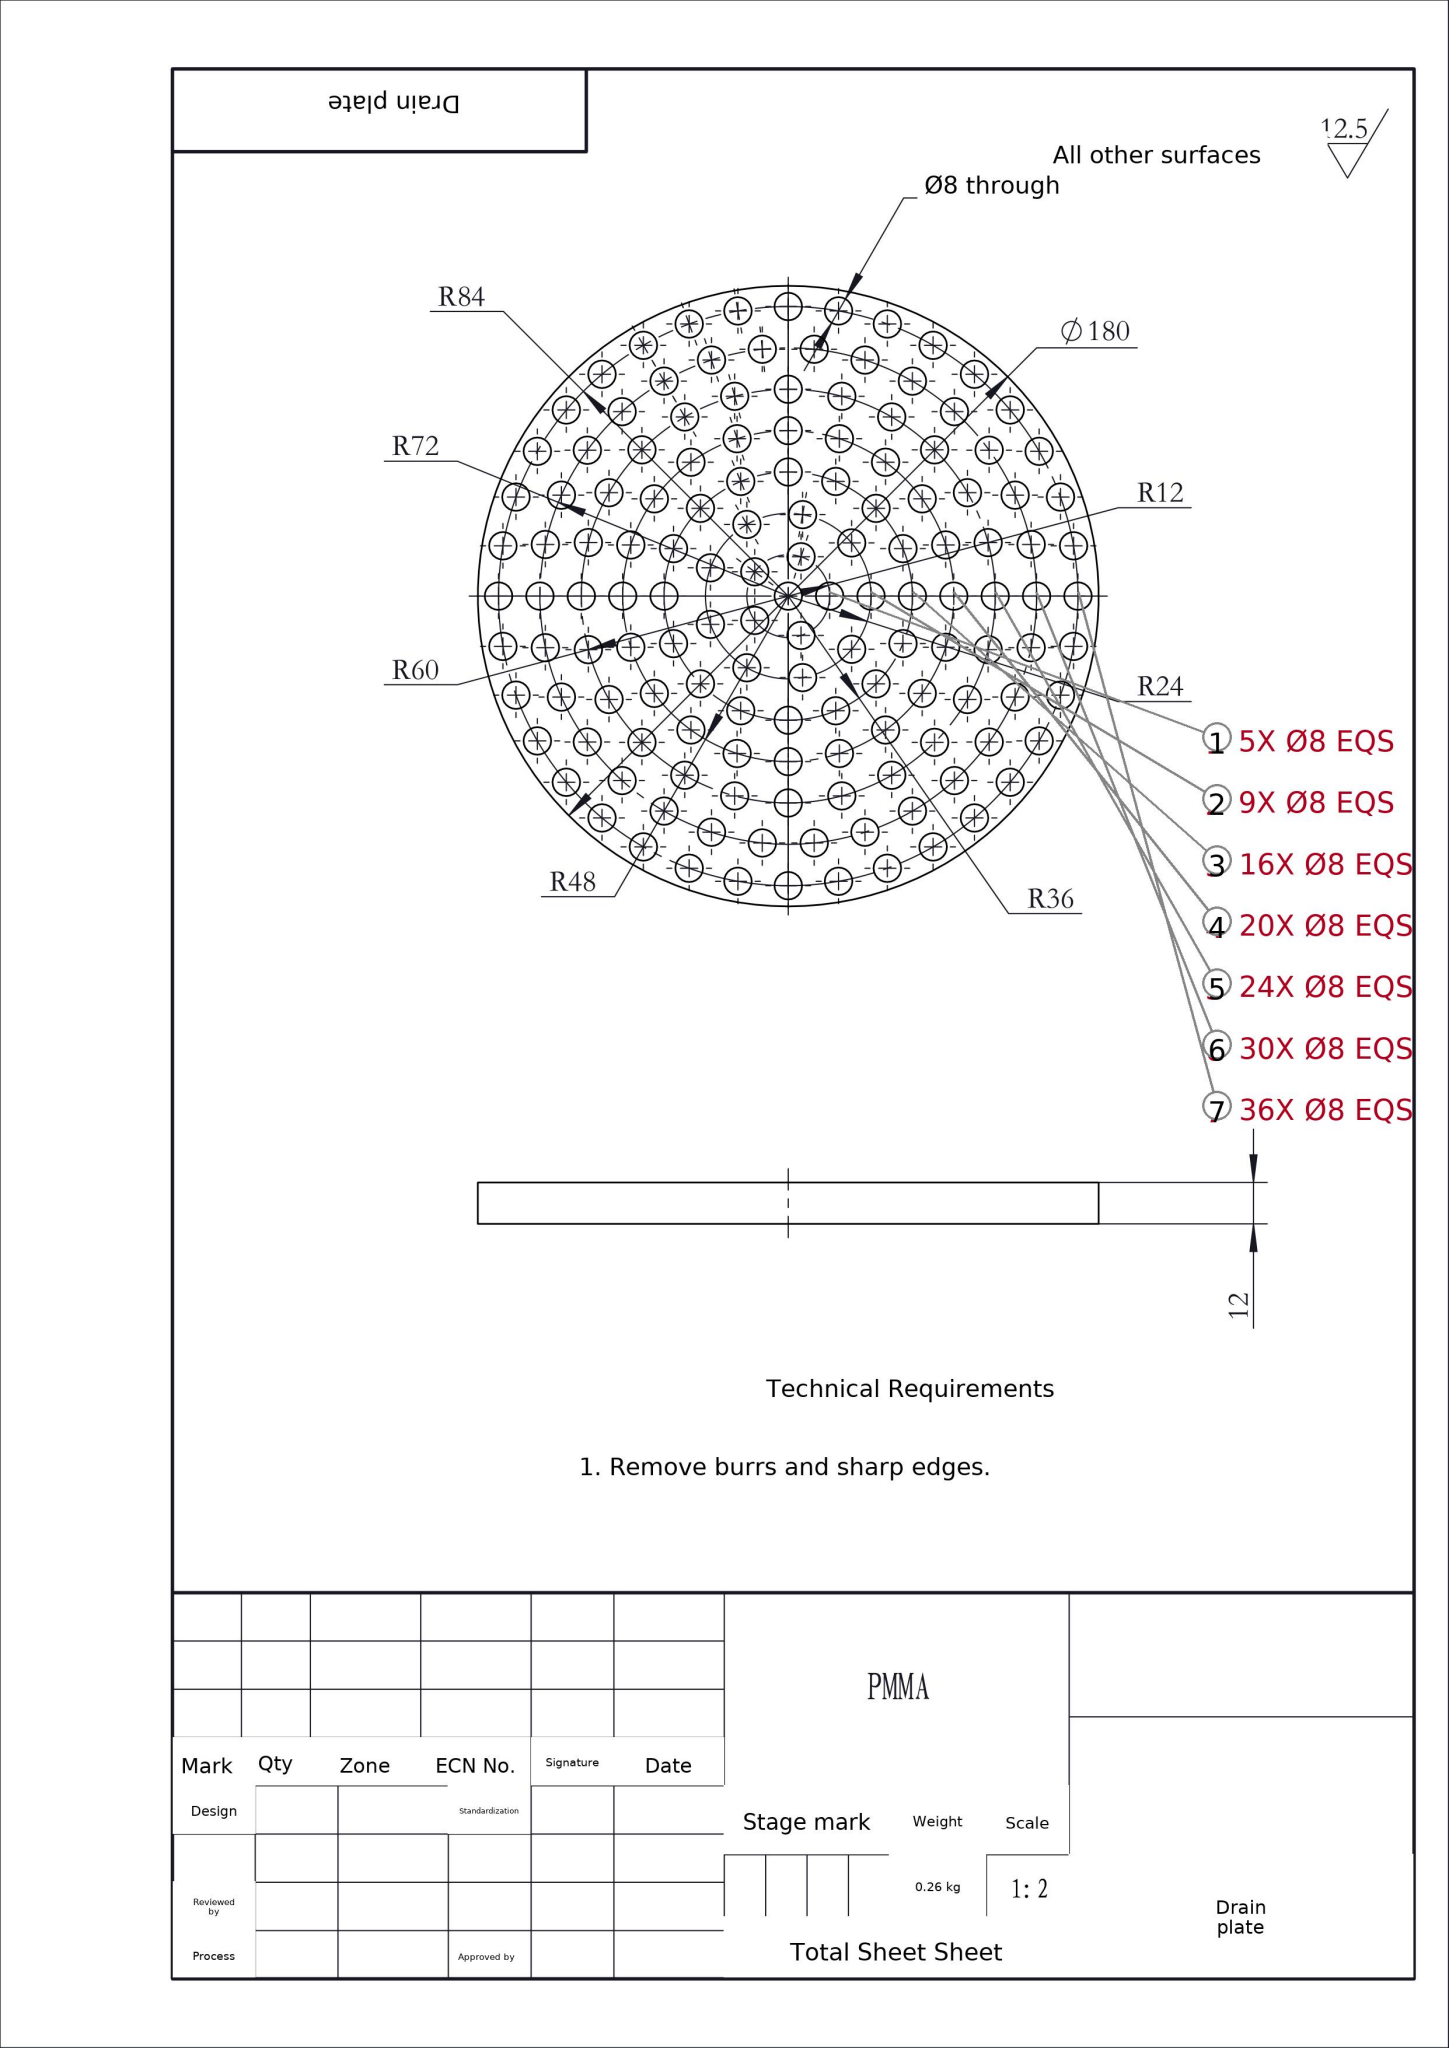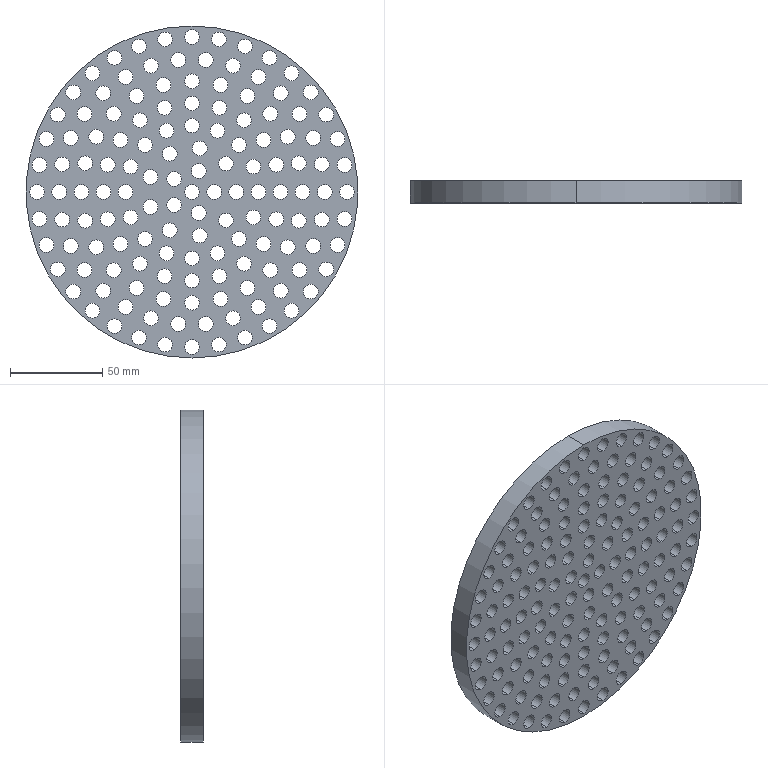Part | SolidWorks | mm | material PMMA | 1 solid | 286 faces | box 180 x 12 x 180 mm | volume 220314 mm3 | cylinder 284 | plane 2 | commonest cylinder face diameters 8 x282 180 x2
build123d program:
from build123d import *

# Parameters (mm, degrees)
SKETCH1_R            = 95
SKETCH1_R_2          = 90
BOSS_EXTRUDE1_DEPTH  = 100
SKETCH2_R            = 90
BOSS_EXTRUDE2_DEPTH  = 8
SKETCH3_R            = 117
SKETCH3_R_2          = 95
SKETCH3_R_3          = 4.25
BOSS_EXTRUDE3_DEPTH  = 12
SKETCH19_R           = 90
SKETCH19_R_2         = 4
BOSS_EXTRUDE20_DEPTH = 6
SKETCH4_R            = 95
SKETCH4_R_2          = 90
BOSS_EXTRUDE4_DEPTH  = 570
SKETCH5_R            = 5
CUT_EXTRUDE2_DEPTH   = 100
SKETCH14_R           = 12.5
CUT_EXTRUDE3_DEPTH   = 12
SKETCH15_R           = 22.5
SKETCH15_R_2         = 12.5
BOSS_EXTRUDE12_DEPTH = 10
SKETCH25_R           = 95
CUT_EXTRUDE15_DEPTH  = 633
SKETCH26_R           = 117
CUT_EXTRUDE16_DEPTH  = 633
CUT_EXTRUDE17_START  = -633
SKETCH27_R           = 117
SKETCH27_R_2         = 90
CUT_EXTRUDE17_DEPTH  = 633
CUT_EXTRUDE18_START  = -633
SKETCH28_R           = 90
CUT_EXTRUDE18_DEPTH  = 633


with BuildPart() as part:
    # Sketch1 → Boss-Extrude1 (new body)
    with BuildSketch(Plane(origin=(0, 0, 0), x_dir=(1, 0, 0), z_dir=(0, 1, 0))):
        with Locations(Location((0, 0, 0), (0, 0, 270))):
            Circle(SKETCH1_R)
        with Locations(Location((0, 0, 0), (0, 0, 270))):
            Circle(SKETCH1_R_2, mode=Mode.SUBTRACT)
    extrude(amount=BOSS_EXTRUDE1_DEPTH)


with BuildPart() as body_2:
    # Sketch2 → Boss-Extrude2 (new body)
    with BuildSketch(Plane(origin=(0, 0, 0), x_dir=(1, 0, 0), z_dir=(0, 1, 0))):
        with Locations(Location((0, 0, 0), (0, 0, 270))):
            Circle(SKETCH2_R)
    extrude(amount=BOSS_EXTRUDE2_DEPTH)

    # Sketch14 → Cut-Extrude3 (cut)
    with BuildSketch(Plane.XZ):
        with Locations(Location((0, -60, 0), (0, 0, 270))):
            Circle(SKETCH14_R)
    extrude(amount=-CUT_EXTRUDE3_DEPTH, mode=Mode.SUBTRACT)


with BuildPart() as body_3:
    # Sketch3 → Boss-Extrude3 (new body)
    with BuildSketch(Plane(origin=(0, 100, 0), x_dir=(1, 0, 0), z_dir=(0, 1, 0))):
        with Locations(Location((0, 0, 0), (0, 0, 270))):
            Circle(SKETCH3_R)
        with Locations(Location((0, 0, 0), (0, 0, 270))):
            Circle(SKETCH3_R_2, mode=Mode.SUBTRACT)
        with Locations(Location((-100.516, 30.358, 0), (0, 0, 270))):
            Circle(SKETCH3_R_3, mode=Mode.SUBTRACT)
        with Locations(Location((-49.609, 92.542, 0), (0, 0, 270))):
            Circle(SKETCH3_R_3, mode=Mode.SUBTRACT)
        with Locations(Location((30.358, 100.516, 0), (0, 0, 270))):
            Circle(SKETCH3_R_3, mode=Mode.SUBTRACT)
        with Locations(Location((92.542, 49.609, 0), (0, 0, 270))):
            Circle(SKETCH3_R_3, mode=Mode.SUBTRACT)
        with Locations(Location((100.516, -30.358, 0), (0, 0, 270))):
            Circle(SKETCH3_R_3, mode=Mode.SUBTRACT)
        with Locations(Location((49.609, -92.542, 0), (0, 0, 270))):
            Circle(SKETCH3_R_3, mode=Mode.SUBTRACT)
        with Locations(Location((-30.358, -100.516, 0), (0, 0, 270))):
            Circle(SKETCH3_R_3, mode=Mode.SUBTRACT)
        with Locations(Location((-92.542, -49.609, 0), (0, 0, 270))):
            Circle(SKETCH3_R_3, mode=Mode.SUBTRACT)
    extrude(amount=-BOSS_EXTRUDE3_DEPTH)


with BuildPart() as body_4:
    # Sketch19 → Boss-Extrude20 (new, symmetric)
    with BuildSketch(Plane(origin=(0, 100, 0), x_dir=(1, 0, 0), z_dir=(0, 1, 0))):
        with Locations(Location((0, 0, 0), (0, 0, 270))):
            Circle(SKETCH19_R)
        with Locations(Location((0, 0, 0), (0, 0, 270))):
            Circle(SKETCH19_R_2, mode=Mode.SUBTRACT)
        with Locations(Location((12, 0, 0), (0, 0, 270))):
            Circle(SKETCH19_R_2, mode=Mode.SUBTRACT)
        with Locations(Location((24, 0, 0), (0, 0, 270))):
            Circle(SKETCH19_R_2, mode=Mode.SUBTRACT)
        with Locations(Location((36, 0, 0), (0, 0, 270))):
            Circle(SKETCH19_R_2, mode=Mode.SUBTRACT)
        with Locations(Location((48, 0, 0), (0, 0, 270))):
            Circle(SKETCH19_R_2, mode=Mode.SUBTRACT)
        with Locations(Location((60, 0, 0), (0, 0, 270))):
            Circle(SKETCH19_R_2, mode=Mode.SUBTRACT)
        with Locations(Location((72, 0, 0), (0, 0, 270))):
            Circle(SKETCH19_R_2, mode=Mode.SUBTRACT)
        with Locations(Location((84, 0, 0), (0, 0, 270))):
            Circle(SKETCH19_R_2, mode=Mode.SUBTRACT)
        with Locations(Location((3.708, -11.413, 0), (0, 0, 270))):
            Circle(SKETCH19_R_2, mode=Mode.SUBTRACT)
        with Locations(Location((-9.708, -7.053, 0), (0, 0, 270))):
            Circle(SKETCH19_R_2, mode=Mode.SUBTRACT)
        with Locations(Location((-9.708, 7.053, 0), (0, 0, 270))):
            Circle(SKETCH19_R_2, mode=Mode.SUBTRACT)
        with Locations(Location((18.385, -15.427, 0), (0, 0, 270))):
            Circle(SKETCH19_R_2, mode=Mode.SUBTRACT)
        with Locations(Location((4.168, -23.635, 0), (0, 0, 270))):
            Circle(SKETCH19_R_2, mode=Mode.SUBTRACT)
        with Locations(Location((-12, -20.785, 0), (0, 0, 270))):
            Circle(SKETCH19_R_2, mode=Mode.SUBTRACT)
        with Locations(Location((-22.553, -8.208, 0), (0, 0, 270))):
            Circle(SKETCH19_R_2, mode=Mode.SUBTRACT)
        with Locations(Location((-22.553, 8.208, 0), (0, 0, 270))):
            Circle(SKETCH19_R_2, mode=Mode.SUBTRACT)
        with Locations(Location((-12, 20.785, 0), (0, 0, 270))):
            Circle(SKETCH19_R_2, mode=Mode.SUBTRACT)
        with Locations(Location((4.168, 23.635, 0), (0, 0, 270))):
            Circle(SKETCH19_R_2, mode=Mode.SUBTRACT)
        with Locations(Location((33.26, -13.777, 0), (0, 0, 270))):
            Circle(SKETCH19_R_2, mode=Mode.SUBTRACT)
        with Locations(Location((25.456, -25.456, 0), (0, 0, 270))):
            Circle(SKETCH19_R_2, mode=Mode.SUBTRACT)
        with Locations(Location((13.777, -33.26, 0), (0, 0, 270))):
            Circle(SKETCH19_R_2, mode=Mode.SUBTRACT)
        with Locations(Location((0, -36, 0), (0, 0, 270))):
            Circle(SKETCH19_R_2, mode=Mode.SUBTRACT)
        with Locations(Location((-13.777, -33.26, 0), (0, 0, 270))):
            Circle(SKETCH19_R_2, mode=Mode.SUBTRACT)
        with Locations(Location((-25.456, -25.456, 0), (0, 0, 270))):
            Circle(SKETCH19_R_2, mode=Mode.SUBTRACT)
        with Locations(Location((-33.26, -13.777, 0), (0, 0, 270))):
            Circle(SKETCH19_R_2, mode=Mode.SUBTRACT)
        with Locations(Location((-36, 0, 0), (0, 0, 270))):
            Circle(SKETCH19_R_2, mode=Mode.SUBTRACT)
        with Locations(Location((-33.26, 13.777, 0), (0, 0, 270))):
            Circle(SKETCH19_R_2, mode=Mode.SUBTRACT)
        with Locations(Location((-25.456, 25.456, 0), (0, 0, 270))):
            Circle(SKETCH19_R_2, mode=Mode.SUBTRACT)
        with Locations(Location((-13.777, 33.26, 0), (0, 0, 270))):
            Circle(SKETCH19_R_2, mode=Mode.SUBTRACT)
        with Locations(Location((45.651, -14.833, 0), (0, 0, 270))):
            Circle(SKETCH19_R_2, mode=Mode.SUBTRACT)
        with Locations(Location((38.833, -28.214, 0), (0, 0, 270))):
            Circle(SKETCH19_R_2, mode=Mode.SUBTRACT)
        with Locations(Location((28.214, -38.833, 0), (0, 0, 270))):
            Circle(SKETCH19_R_2, mode=Mode.SUBTRACT)
        with Locations(Location((14.833, -45.651, 0), (0, 0, 270))):
            Circle(SKETCH19_R_2, mode=Mode.SUBTRACT)
        with Locations(Location((0, -48, 0), (0, 0, 270))):
            Circle(SKETCH19_R_2, mode=Mode.SUBTRACT)
        with Locations(Location((-14.833, -45.651, 0), (0, 0, 270))):
            Circle(SKETCH19_R_2, mode=Mode.SUBTRACT)
        with Locations(Location((-28.214, -38.833, 0), (0, 0, 270))):
            Circle(SKETCH19_R_2, mode=Mode.SUBTRACT)
        with Locations(Location((-38.833, -28.214, 0), (0, 0, 270))):
            Circle(SKETCH19_R_2, mode=Mode.SUBTRACT)
        with Locations(Location((-45.651, -14.833, 0), (0, 0, 270))):
            Circle(SKETCH19_R_2, mode=Mode.SUBTRACT)
        with Locations(Location((-48, 0, 0), (0, 0, 270))):
            Circle(SKETCH19_R_2, mode=Mode.SUBTRACT)
        with Locations(Location((-45.651, 14.833, 0), (0, 0, 270))):
            Circle(SKETCH19_R_2, mode=Mode.SUBTRACT)
        with Locations(Location((-38.833, 28.214, 0), (0, 0, 270))):
            Circle(SKETCH19_R_2, mode=Mode.SUBTRACT)
        with Locations(Location((-28.214, 38.833, 0), (0, 0, 270))):
            Circle(SKETCH19_R_2, mode=Mode.SUBTRACT)
        with Locations(Location((-14.833, 45.651, 0), (0, 0, 270))):
            Circle(SKETCH19_R_2, mode=Mode.SUBTRACT)
        with Locations(Location((0, 48, 0), (0, 0, 270))):
            Circle(SKETCH19_R_2, mode=Mode.SUBTRACT)
        with Locations(Location((14.833, 45.651, 0), (0, 0, 270))):
            Circle(SKETCH19_R_2, mode=Mode.SUBTRACT)
        with Locations(Location((28.214, 38.833, 0), (0, 0, 270))):
            Circle(SKETCH19_R_2, mode=Mode.SUBTRACT)
        with Locations(Location((38.833, 28.214, 0), (0, 0, 270))):
            Circle(SKETCH19_R_2, mode=Mode.SUBTRACT)
        with Locations(Location((45.651, 14.833, 0), (0, 0, 270))):
            Circle(SKETCH19_R_2, mode=Mode.SUBTRACT)
        with Locations(Location((57.956, -15.529, 0), (0, 0, 270))):
            Circle(SKETCH19_R_2, mode=Mode.SUBTRACT)
        with Locations(Location((51.962, -30, 0), (0, 0, 270))):
            Circle(SKETCH19_R_2, mode=Mode.SUBTRACT)
        with Locations(Location((42.426, -42.426, 0), (0, 0, 270))):
            Circle(SKETCH19_R_2, mode=Mode.SUBTRACT)
        with Locations(Location((30, -51.962, 0), (0, 0, 270))):
            Circle(SKETCH19_R_2, mode=Mode.SUBTRACT)
        with Locations(Location((15.529, -57.956, 0), (0, 0, 270))):
            Circle(SKETCH19_R_2, mode=Mode.SUBTRACT)
        with Locations(Location((0, -60, 0), (0, 0, 270))):
            Circle(SKETCH19_R_2, mode=Mode.SUBTRACT)
        with Locations(Location((-15.529, -57.956, 0), (0, 0, 270))):
            Circle(SKETCH19_R_2, mode=Mode.SUBTRACT)
        with Locations(Location((-30, -51.962, 0), (0, 0, 270))):
            Circle(SKETCH19_R_2, mode=Mode.SUBTRACT)
        with Locations(Location((-42.426, -42.426, 0), (0, 0, 270))):
            Circle(SKETCH19_R_2, mode=Mode.SUBTRACT)
        with Locations(Location((-51.962, -30, 0), (0, 0, 270))):
            Circle(SKETCH19_R_2, mode=Mode.SUBTRACT)
        with Locations(Location((-57.956, -15.529, 0), (0, 0, 270))):
            Circle(SKETCH19_R_2, mode=Mode.SUBTRACT)
        with Locations(Location((-60, 0, 0), (0, 0, 270))):
            Circle(SKETCH19_R_2, mode=Mode.SUBTRACT)
        with Locations(Location((-57.956, 15.529, 0), (0, 0, 270))):
            Circle(SKETCH19_R_2, mode=Mode.SUBTRACT)
        with Locations(Location((-51.962, 30, 0), (0, 0, 270))):
            Circle(SKETCH19_R_2, mode=Mode.SUBTRACT)
        with Locations(Location((-42.426, 42.426, 0), (0, 0, 270))):
            Circle(SKETCH19_R_2, mode=Mode.SUBTRACT)
        with Locations(Location((-30, 51.962, 0), (0, 0, 270))):
            Circle(SKETCH19_R_2, mode=Mode.SUBTRACT)
        with Locations(Location((-15.529, 57.956, 0), (0, 0, 270))):
            Circle(SKETCH19_R_2, mode=Mode.SUBTRACT)
        with Locations(Location((0, 60, 0), (0, 0, 270))):
            Circle(SKETCH19_R_2, mode=Mode.SUBTRACT)
        with Locations(Location((15.529, 57.956, 0), (0, 0, 270))):
            Circle(SKETCH19_R_2, mode=Mode.SUBTRACT)
        with Locations(Location((30, 51.962, 0), (0, 0, 270))):
            Circle(SKETCH19_R_2, mode=Mode.SUBTRACT)
        with Locations(Location((42.426, 42.426, 0), (0, 0, 270))):
            Circle(SKETCH19_R_2, mode=Mode.SUBTRACT)
        with Locations(Location((51.962, 30, 0), (0, 0, 270))):
            Circle(SKETCH19_R_2, mode=Mode.SUBTRACT)
        with Locations(Location((57.956, 15.529, 0), (0, 0, 270))):
            Circle(SKETCH19_R_2, mode=Mode.SUBTRACT)
        with Locations(Location((70.427, -14.97, 0), (0, 0, 270))):
            Circle(SKETCH19_R_2, mode=Mode.SUBTRACT)
        with Locations(Location((65.775, -29.285, 0), (0, 0, 270))):
            Circle(SKETCH19_R_2, mode=Mode.SUBTRACT)
        with Locations(Location((58.249, -42.321, 0), (0, 0, 270))):
            Circle(SKETCH19_R_2, mode=Mode.SUBTRACT)
        with Locations(Location((48.177, -53.506, 0), (0, 0, 270))):
            Circle(SKETCH19_R_2, mode=Mode.SUBTRACT)
        with Locations(Location((36, -62.354, 0), (0, 0, 270))):
            Circle(SKETCH19_R_2, mode=Mode.SUBTRACT)
        with Locations(Location((22.249, -68.476, 0), (0, 0, 270))):
            Circle(SKETCH19_R_2, mode=Mode.SUBTRACT)
        with Locations(Location((7.526, -71.606, 0), (0, 0, 270))):
            Circle(SKETCH19_R_2, mode=Mode.SUBTRACT)
        with Locations(Location((-7.526, -71.606, 0), (0, 0, 270))):
            Circle(SKETCH19_R_2, mode=Mode.SUBTRACT)
        with Locations(Location((-22.249, -68.476, 0), (0, 0, 270))):
            Circle(SKETCH19_R_2, mode=Mode.SUBTRACT)
        with Locations(Location((-36, -62.354, 0), (0, 0, 270))):
            Circle(SKETCH19_R_2, mode=Mode.SUBTRACT)
        with Locations(Location((-48.177, -53.506, 0), (0, 0, 270))):
            Circle(SKETCH19_R_2, mode=Mode.SUBTRACT)
        with Locations(Location((-58.249, -42.321, 0), (0, 0, 270))):
            Circle(SKETCH19_R_2, mode=Mode.SUBTRACT)
        with Locations(Location((-65.775, -29.285, 0), (0, 0, 270))):
            Circle(SKETCH19_R_2, mode=Mode.SUBTRACT)
        with Locations(Location((-70.427, -14.97, 0), (0, 0, 270))):
            Circle(SKETCH19_R_2, mode=Mode.SUBTRACT)
        with Locations(Location((-72, 0, 0), (0, 0, 270))):
            Circle(SKETCH19_R_2, mode=Mode.SUBTRACT)
        with Locations(Location((-70.427, 14.97, 0), (0, 0, 270))):
            Circle(SKETCH19_R_2, mode=Mode.SUBTRACT)
        with Locations(Location((-65.775, 29.285, 0), (0, 0, 270))):
            Circle(SKETCH19_R_2, mode=Mode.SUBTRACT)
        with Locations(Location((-58.249, 42.321, 0), (0, 0, 270))):
            Circle(SKETCH19_R_2, mode=Mode.SUBTRACT)
        with Locations(Location((-48.177, 53.506, 0), (0, 0, 270))):
            Circle(SKETCH19_R_2, mode=Mode.SUBTRACT)
        with Locations(Location((-36, 62.354, 0), (0, 0, 270))):
            Circle(SKETCH19_R_2, mode=Mode.SUBTRACT)
        with Locations(Location((-22.249, 68.476, 0), (0, 0, 270))):
            Circle(SKETCH19_R_2, mode=Mode.SUBTRACT)
        with Locations(Location((-7.526, 71.606, 0), (0, 0, 270))):
            Circle(SKETCH19_R_2, mode=Mode.SUBTRACT)
        with Locations(Location((7.526, 71.606, 0), (0, 0, 270))):
            Circle(SKETCH19_R_2, mode=Mode.SUBTRACT)
        with Locations(Location((22.249, 68.476, 0), (0, 0, 270))):
            Circle(SKETCH19_R_2, mode=Mode.SUBTRACT)
        with Locations(Location((36, 62.354, 0), (0, 0, 270))):
            Circle(SKETCH19_R_2, mode=Mode.SUBTRACT)
        with Locations(Location((48.177, 53.506, 0), (0, 0, 270))):
            Circle(SKETCH19_R_2, mode=Mode.SUBTRACT)
        with Locations(Location((58.249, 42.321, 0), (0, 0, 270))):
            Circle(SKETCH19_R_2, mode=Mode.SUBTRACT)
        with Locations(Location((65.775, 29.285, 0), (0, 0, 270))):
            Circle(SKETCH19_R_2, mode=Mode.SUBTRACT)
        with Locations(Location((70.427, 14.97, 0), (0, 0, 270))):
            Circle(SKETCH19_R_2, mode=Mode.SUBTRACT)
        with Locations(Location((82.724, -14.586, 0), (0, 0, 270))):
            Circle(SKETCH19_R_2, mode=Mode.SUBTRACT)
        with Locations(Location((78.934, -28.73, 0), (0, 0, 270))):
            Circle(SKETCH19_R_2, mode=Mode.SUBTRACT)
        with Locations(Location((72.746, -42, 0), (0, 0, 270))):
            Circle(SKETCH19_R_2, mode=Mode.SUBTRACT)
        with Locations(Location((64.348, -53.994, 0), (0, 0, 270))):
            Circle(SKETCH19_R_2, mode=Mode.SUBTRACT)
        with Locations(Location((53.994, -64.348, 0), (0, 0, 270))):
            Circle(SKETCH19_R_2, mode=Mode.SUBTRACT)
        with Locations(Location((42, -72.746, 0), (0, 0, 270))):
            Circle(SKETCH19_R_2, mode=Mode.SUBTRACT)
        with Locations(Location((28.73, -78.934, 0), (0, 0, 270))):
            Circle(SKETCH19_R_2, mode=Mode.SUBTRACT)
        with Locations(Location((14.586, -82.724, 0), (0, 0, 270))):
            Circle(SKETCH19_R_2, mode=Mode.SUBTRACT)
        with Locations(Location((0, -84, 0), (0, 0, 270))):
            Circle(SKETCH19_R_2, mode=Mode.SUBTRACT)
        with Locations(Location((-14.586, -82.724, 0), (0, 0, 270))):
            Circle(SKETCH19_R_2, mode=Mode.SUBTRACT)
        with Locations(Location((-28.73, -78.934, 0), (0, 0, 270))):
            Circle(SKETCH19_R_2, mode=Mode.SUBTRACT)
        with Locations(Location((-42, -72.746, 0), (0, 0, 270))):
            Circle(SKETCH19_R_2, mode=Mode.SUBTRACT)
        with Locations(Location((-53.994, -64.348, 0), (0, 0, 270))):
            Circle(SKETCH19_R_2, mode=Mode.SUBTRACT)
        with Locations(Location((-64.348, -53.994, 0), (0, 0, 270))):
            Circle(SKETCH19_R_2, mode=Mode.SUBTRACT)
        with Locations(Location((-72.746, -42, 0), (0, 0, 270))):
            Circle(SKETCH19_R_2, mode=Mode.SUBTRACT)
        with Locations(Location((-78.934, -28.73, 0), (0, 0, 270))):
            Circle(SKETCH19_R_2, mode=Mode.SUBTRACT)
        with Locations(Location((-82.724, -14.586, 0), (0, 0, 270))):
            Circle(SKETCH19_R_2, mode=Mode.SUBTRACT)
        with Locations(Location((-84, 0, 0), (0, 0, 270))):
            Circle(SKETCH19_R_2, mode=Mode.SUBTRACT)
        with Locations(Location((-82.724, 14.586, 0), (0, 0, 270))):
            Circle(SKETCH19_R_2, mode=Mode.SUBTRACT)
        with Locations(Location((-78.934, 28.73, 0), (0, 0, 270))):
            Circle(SKETCH19_R_2, mode=Mode.SUBTRACT)
        with Locations(Location((-72.746, 42, 0), (0, 0, 270))):
            Circle(SKETCH19_R_2, mode=Mode.SUBTRACT)
        with Locations(Location((-64.348, 53.994, 0), (0, 0, 270))):
            Circle(SKETCH19_R_2, mode=Mode.SUBTRACT)
        with Locations(Location((-53.994, 64.348, 0), (0, 0, 270))):
            Circle(SKETCH19_R_2, mode=Mode.SUBTRACT)
        with Locations(Location((-42, 72.746, 0), (0, 0, 270))):
            Circle(SKETCH19_R_2, mode=Mode.SUBTRACT)
        with Locations(Location((-28.73, 78.934, 0), (0, 0, 270))):
            Circle(SKETCH19_R_2, mode=Mode.SUBTRACT)
        with Locations(Location((-14.586, 82.724, 0), (0, 0, 270))):
            Circle(SKETCH19_R_2, mode=Mode.SUBTRACT)
        with Locations(Location((0, 84, 0), (0, 0, 270))):
            Circle(SKETCH19_R_2, mode=Mode.SUBTRACT)
        with Locations(Location((14.586, 82.724, 0), (0, 0, 270))):
            Circle(SKETCH19_R_2, mode=Mode.SUBTRACT)
        with Locations(Location((28.73, 78.934, 0), (0, 0, 270))):
            Circle(SKETCH19_R_2, mode=Mode.SUBTRACT)
        with Locations(Location((42, 72.746, 0), (0, 0, 270))):
            Circle(SKETCH19_R_2, mode=Mode.SUBTRACT)
        with Locations(Location((53.994, 64.348, 0), (0, 0, 270))):
            Circle(SKETCH19_R_2, mode=Mode.SUBTRACT)
        with Locations(Location((64.348, 53.994, 0), (0, 0, 270))):
            Circle(SKETCH19_R_2, mode=Mode.SUBTRACT)
        with Locations(Location((72.746, 42, 0), (0, 0, 270))):
            Circle(SKETCH19_R_2, mode=Mode.SUBTRACT)
        with Locations(Location((78.934, 28.73, 0), (0, 0, 270))):
            Circle(SKETCH19_R_2, mode=Mode.SUBTRACT)
        with Locations(Location((82.724, 14.586, 0), (0, 0, 270))):
            Circle(SKETCH19_R_2, mode=Mode.SUBTRACT)
        with Locations(Location((0, 36, 0), (0, 0, 270))):
            Circle(SKETCH19_R_2, mode=Mode.SUBTRACT)
        with Locations(Location((13.777, 33.26, 0), (0, 0, 270))):
            Circle(SKETCH19_R_2, mode=Mode.SUBTRACT)
        with Locations(Location((25.456, 25.456, 0), (0, 0, 270))):
            Circle(SKETCH19_R_2, mode=Mode.SUBTRACT)
        with Locations(Location((33.26, 13.777, 0), (0, 0, 270))):
            Circle(SKETCH19_R_2, mode=Mode.SUBTRACT)
        with Locations(Location((18.385, 15.427, 0), (0, 0, 270))):
            Circle(SKETCH19_R_2, mode=Mode.SUBTRACT)
        with Locations(Location((3.708, 11.413, 0), (0, 0, 270))):
            Circle(SKETCH19_R_2, mode=Mode.SUBTRACT)
    extrude(amount=BOSS_EXTRUDE20_DEPTH, both=True)


with BuildPart() as body_5:
    # Mirror1: mirrored copy
    add(body_3.part.mirror(Plane.ZX.offset(103)))

    # Sketch26 → Cut-Extrude16 (cut)
    with BuildSketch(Plane.XZ.offset(-106)):
        with Locations(Location((0, 0, 0), (0, 0, 90))):
            Circle(SKETCH26_R)
    extrude(amount=-CUT_EXTRUDE16_DEPTH, mode=Mode.SUBTRACT)


with BuildPart() as body_6:
    # Sketch4 → Boss-Extrude4 (new body)
    with BuildSketch(Plane.XZ.offset(-106)):
        with Locations(Location((0, 0, 0), (0, 0, 90))):
            Circle(SKETCH4_R)
        with Locations(Location((0, 0, 0), (0, 0, 90))):
            Circle(SKETCH4_R_2, mode=Mode.SUBTRACT)
    extrude(amount=-BOSS_EXTRUDE4_DEPTH)


with BuildPart() as cut_extrude2_tool:
    # Sketch5 → Cut-Extrude2 (new body)
    with BuildSketch(Plane(origin=(0, 0, 0), x_dir=(0, 0, -1), z_dir=(1, 0, 0))):
        with Locations(Location((0, 556, 0), (0, 0, 180))):
            Circle(SKETCH5_R)
        with Locations(Location((0, 139.5, 0), (0, 0, 180))):
            Circle(SKETCH5_R)
        with Locations(Location((0, 80, 0), (0, 0, 180))):
            Circle(SKETCH5_R)
        with Locations(Location((0, 239.5, 0), (0, 0, 180))):
            Circle(SKETCH5_R)
    extrude(amount=CUT_EXTRUDE2_DEPTH)


with BuildPart() as part_1:
    add(part.part)

    # Cut-Extrude2: cut by cut_extrude2_tool
    add(cut_extrude2_tool.part, mode=Mode.SUBTRACT)


    add(body_2.part)  # Boss-Extrude12 merges body 2
    # Sketch15 → Boss-Extrude12 (add)
    with BuildSketch(Plane.XZ):
        with Locations(Location((0, -60, 0), (0, 0, 90))):
            Circle(SKETCH15_R)
        with Locations(Location((0, -60, 0), (0, 0, 270))):
            Circle(SKETCH15_R_2, mode=Mode.SUBTRACT)
    extrude(amount=BOSS_EXTRUDE12_DEPTH)


with BuildPart() as body_6_1:
    add(body_6.part)

    # Cut-Extrude2: cut by cut_extrude2_tool
    add(cut_extrude2_tool.part, mode=Mode.SUBTRACT)

    # Sketch25 → Cut-Extrude15 (cut)
    with BuildSketch(Plane.XZ.offset(-106)):
        with Locations(Location((0, 0, 0), (0, 0, 90))):
            Circle(SKETCH25_R)
    extrude(amount=-CUT_EXTRUDE15_DEPTH, mode=Mode.SUBTRACT)


with BuildPart() as cut_extrude17_tool:
    # Sketch27 → Cut-Extrude17 (new body)
    with BuildSketch(Plane(origin=(0, 100, 0), x_dir=(1, 0, 0), z_dir=(0, 1, 0)).offset(CUT_EXTRUDE17_START)):
        Circle(SKETCH27_R)
        with Locations(Location((0, 0, 0), (0, 0, 270))):
            Circle(SKETCH27_R_2, mode=Mode.SUBTRACT)
    extrude(amount=CUT_EXTRUDE17_DEPTH)


with BuildPart() as part_2:
    add(part_1.part)

    # Cut-Extrude17: cut by cut_extrude17_tool
    add(cut_extrude17_tool.part, mode=Mode.SUBTRACT)

    # Sketch28 → Cut-Extrude18 (cut)
    with BuildSketch(Plane(origin=(0, 8, 0), x_dir=(1, 0, 0), z_dir=(0, 1, 0)).offset(CUT_EXTRUDE18_START)):
        with Locations(Location((0, 0, 0), (0, 0, 270))):
            Circle(SKETCH28_R)
    extrude(amount=CUT_EXTRUDE18_DEPTH, mode=Mode.SUBTRACT)


with BuildPart() as body_3_1:
    add(body_3.part)

    # Cut-Extrude17: cut by cut_extrude17_tool
    add(cut_extrude17_tool.part, mode=Mode.SUBTRACT)


solid = body_4.part